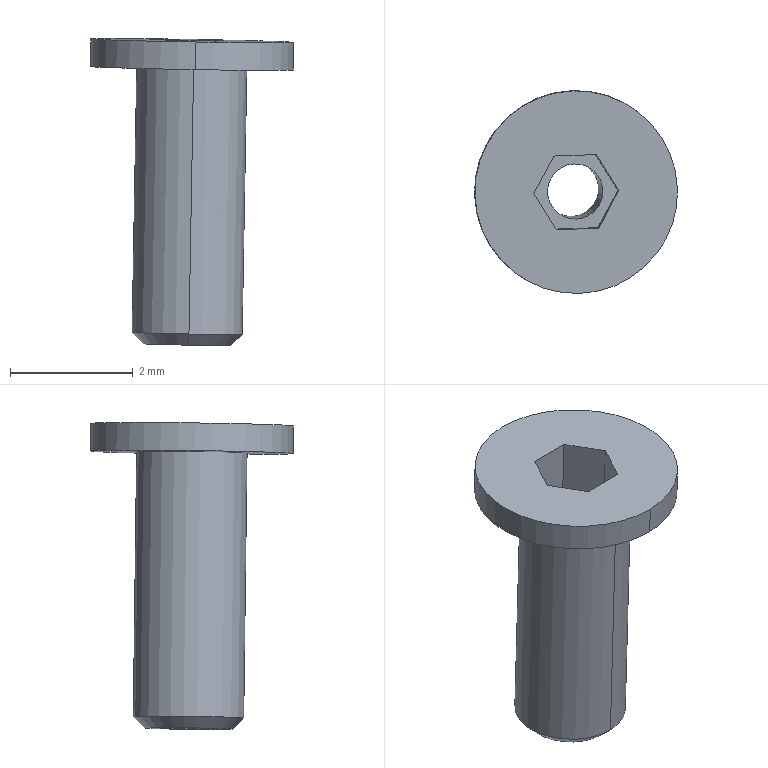Component | SolidWorks | 00-VacuumSuctionCupAssembly-1_10-SuctionCupAirHoleScrew-12 | 1 solid | 18 faces | box 3.31 x 3.31 x 5 mm | volume 12 mm3 | plane 10 | cylinder 6 | cone 2 | commonest cylinder face diameters 0.9 x2 1.8 x2 3.3 x2
STEP:
#1=COLOUR_RGB('',0.7922,0.8196,0.9333);
#2=FILL_AREA_STYLE_COLOUR('',#1);
#3=FILL_AREA_STYLE('',(#2));
#4=SURFACE_STYLE_FILL_AREA(#3);
#5=SURFACE_SIDE_STYLE('',(#4));
#6=SURFACE_STYLE_USAGE(.BOTH.,#5);
#7=PRESENTATION_STYLE_ASSIGNMENT((#6));
#8=CARTESIAN_POINT('',(2.26,5.23,2.116));
#9=VERTEX_POINT('',#8);
#10=CARTESIAN_POINT('',(2.258,5.286,2.117));
#11=VERTEX_POINT('',#10);
#12=CARTESIAN_POINT('',(2.259,5.258,2.116));
#13=DIRECTION('',(-0.01745,0.01259,-0.9998));
#14=DIRECTION('',(0.03309,-0.9994,-0.01316));
#15=AXIS2_PLACEMENT_3D('',#12,#13,#14);
#16=CIRCLE('',#15,0.02819);
#17=EDGE_CURVE('',#9,#11,#16,.T.);
#18=ORIENTED_EDGE('',*,*,#17,.F.);
#19=CARTESIAN_POINT('',(2.26,5.223,2.123));
#20=VERTEX_POINT('',#19);
#21=CARTESIAN_POINT('',(2.26,5.23,2.116));
#22=DIRECTION('',(0.03574,-0.7156,0.6976));
#23=VECTOR('',#22,39.37);
#24=LINE('',#21,#23);
#25=EDGE_CURVE('',#9,#20,#24,.T.);
#26=ORIENTED_EDGE('',*,*,#25,.T.);
#27=CARTESIAN_POINT('',(2.258,5.293,2.124));
#28=VERTEX_POINT('',#27);
#29=CARTESIAN_POINT('',(2.259,5.258,2.124));
#30=DIRECTION('',(0.01745,-0.01259,0.9998));
#31=DIRECTION('',(0.03309,-0.9994,-0.01316));
#32=AXIS2_PLACEMENT_3D('',#29,#30,#31);
#33=CIRCLE('',#32,0.03543);
#34=EDGE_CURVE('',#28,#20,#33,.T.);
#35=ORIENTED_EDGE('',*,*,#34,.F.);
#36=CARTESIAN_POINT('',(2.258,5.286,2.117));
#37=DIRECTION('',(-0.01106,0.6978,0.7162));
#38=VECTOR('',#37,39.37);
#39=LINE('',#36,#38);
#40=EDGE_CURVE('',#11,#28,#39,.T.);
#41=ORIENTED_EDGE('',*,*,#40,.F.);
#42=EDGE_LOOP('',(#18,#26,#35,#41));
#43=FACE_OUTER_BOUND('',#42,.T.);
#44=CARTESIAN_POINT('',(2.259,5.258,2.116));
#45=DIRECTION('',(0.01745,-0.01259,0.9998));
#46=DIRECTION('',(-0.03309,0.9994,0.01316));
#47=AXIS2_PLACEMENT_3D('',#44,#45,#46);
#48=CONICAL_SURFACE('',#47,0.02819,0.7854);
#49=ADVANCED_FACE('',(#43),#48,.T.);
#50=CARTESIAN_POINT('',(2.262,5.238,2.276));
#51=VERTEX_POINT('',#50);
#52=CARTESIAN_POINT('',(2.261,5.274,2.276));
#53=VERTEX_POINT('',#52);
#54=CARTESIAN_POINT('',(2.262,5.256,2.276));
#55=DIRECTION('',(0.01745,-0.01259,0.9998));
#56=DIRECTION('',(-0.03309,0.9994,0.01316));
#57=AXIS2_PLACEMENT_3D('',#54,#55,#56);
#58=CIRCLE('',#57,0.01772);
#59=EDGE_CURVE('',#51,#53,#58,.T.);
#60=ORIENTED_EDGE('',*,*,#59,.T.);
#61=CARTESIAN_POINT('',(2.258,5.276,2.117));
#62=VERTEX_POINT('',#61);
#63=CARTESIAN_POINT('',(2.258,5.276,2.117));
#64=DIRECTION('',(-0.01745,0.01259,-0.9998));
#65=VECTOR('',#64,39.37);
#66=LINE('',#63,#65);
#67=EDGE_CURVE('',#53,#62,#66,.T.);
#68=ORIENTED_EDGE('',*,*,#67,.T.);
#69=CARTESIAN_POINT('',(2.26,5.24,2.116));
#70=VERTEX_POINT('',#69);
#71=CARTESIAN_POINT('',(2.259,5.258,2.116));
#72=DIRECTION('',(-0.01745,0.01259,-0.9998));
#73=DIRECTION('',(0.03309,-0.9994,-0.01316));
#74=AXIS2_PLACEMENT_3D('',#71,#72,#73);
#75=CIRCLE('',#74,0.01772);
#76=EDGE_CURVE('',#62,#70,#75,.T.);
#77=ORIENTED_EDGE('',*,*,#76,.T.);
#78=CARTESIAN_POINT('',(2.26,5.24,2.116));
#79=DIRECTION('',(-0.01745,0.01259,-0.9998));
#80=VECTOR('',#79,39.37);
#81=LINE('',#78,#80);
#82=EDGE_CURVE('',#51,#70,#81,.T.);
#83=ORIENTED_EDGE('',*,*,#82,.F.);
#84=EDGE_LOOP('',(#60,#68,#77,#83));
#85=FACE_OUTER_BOUND('',#84,.T.);
#86=CARTESIAN_POINT('',(2.259,5.258,2.116));
#87=DIRECTION('',(-0.01745,0.01259,-0.9998));
#88=DIRECTION('',(0.03309,-0.9994,-0.01316));
#89=AXIS2_PLACEMENT_3D('',#86,#87,#88);
#90=CYLINDRICAL_SURFACE('',#89,0.01772);
#91=ADVANCED_FACE('',(#85),#90,.F.);
#92=ORIENTED_EDGE('',*,*,#34,.T.);
#93=CARTESIAN_POINT('',(2.263,5.221,2.293));
#94=VERTEX_POINT('',#93);
#95=CARTESIAN_POINT('',(2.26,5.223,2.116));
#96=DIRECTION('',(0.01745,-0.01259,0.9998));
#97=VECTOR('',#96,39.37);
#98=LINE('',#95,#97);
#99=EDGE_CURVE('',#20,#94,#98,.T.);
#100=ORIENTED_EDGE('',*,*,#99,.T.);
#101=CARTESIAN_POINT('',(2.261,5.291,2.294));
#102=VERTEX_POINT('',#101);
#103=CARTESIAN_POINT('',(2.262,5.256,2.293));
#104=DIRECTION('',(-0.01745,0.01259,-0.9998));
#105=DIRECTION('',(0.03309,-0.9994,-0.01316));
#106=AXIS2_PLACEMENT_3D('',#103,#104,#105);
#107=CIRCLE('',#106,0.03543);
#108=EDGE_CURVE('',#94,#102,#107,.T.);
#109=ORIENTED_EDGE('',*,*,#108,.T.);
#110=CARTESIAN_POINT('',(2.258,5.294,2.117));
#111=DIRECTION('',(0.01745,-0.01259,0.9998));
#112=VECTOR('',#111,39.37);
#113=LINE('',#110,#112);
#114=EDGE_CURVE('',#28,#102,#113,.T.);
#115=ORIENTED_EDGE('',*,*,#114,.F.);
#116=EDGE_LOOP('',(#92,#100,#109,#115));
#117=FACE_OUTER_BOUND('',#116,.T.);
#118=CARTESIAN_POINT('',(2.259,5.258,2.116));
#119=DIRECTION('',(0.01745,-0.01259,0.9998));
#120=DIRECTION('',(-0.03309,0.9994,0.01316));
#121=AXIS2_PLACEMENT_3D('',#118,#119,#120);
#122=CYLINDRICAL_SURFACE('',#121,0.03543);
#123=ADVANCED_FACE('',(#117),#122,.T.);
#124=CARTESIAN_POINT('',(2.26,5.321,2.294));
#125=VERTEX_POINT('',#124);
#126=CARTESIAN_POINT('',(2.264,5.191,2.293));
#127=VERTEX_POINT('',#126);
#128=CARTESIAN_POINT('',(2.262,5.256,2.293));
#129=DIRECTION('',(0.01745,-0.01259,0.9998));
#130=DIRECTION('',(-0.03309,0.9994,0.01316));
#131=AXIS2_PLACEMENT_3D('',#128,#129,#130);
#132=CIRCLE('',#131,0.06496);
#133=EDGE_CURVE('',#125,#127,#132,.T.);
#134=ORIENTED_EDGE('',*,*,#133,.T.);
#135=CARTESIAN_POINT('',(2.264,5.191,2.31));
#136=VERTEX_POINT('',#135);
#137=CARTESIAN_POINT('',(2.264,5.191,2.293));
#138=DIRECTION('',(0.01745,-0.01259,0.9998));
#139=VECTOR('',#138,39.37);
#140=LINE('',#137,#139);
#141=EDGE_CURVE('',#127,#136,#140,.T.);
#142=ORIENTED_EDGE('',*,*,#141,.T.);
#143=CARTESIAN_POINT('',(2.26,5.321,2.312));
#144=VERTEX_POINT('',#143);
#145=CARTESIAN_POINT('',(2.262,5.256,2.311));
#146=DIRECTION('',(0.01745,-0.01259,0.9998));
#147=DIRECTION('',(-0.03309,0.9994,0.01316));
#148=AXIS2_PLACEMENT_3D('',#145,#146,#147);
#149=CIRCLE('',#148,0.06496);
#150=EDGE_CURVE('',#144,#136,#149,.T.);
#151=ORIENTED_EDGE('',*,*,#150,.F.);
#152=CARTESIAN_POINT('',(2.26,5.321,2.294));
#153=DIRECTION('',(0.01745,-0.01259,0.9998));
#154=VECTOR('',#153,39.37);
#155=LINE('',#152,#154);
#156=EDGE_CURVE('',#125,#144,#155,.T.);
#157=ORIENTED_EDGE('',*,*,#156,.F.);
#158=EDGE_LOOP('',(#134,#142,#151,#157));
#159=FACE_OUTER_BOUND('',#158,.T.);
#160=CARTESIAN_POINT('',(2.262,5.256,2.293));
#161=DIRECTION('',(0.01745,-0.01259,0.9998));
#162=DIRECTION('',(-0.03309,0.9994,0.01316));
#163=AXIS2_PLACEMENT_3D('',#160,#161,#162);
#164=CYLINDRICAL_SURFACE('',#163,0.06496);
#165=ADVANCED_FACE('',(#159),#164,.T.);
#166=ORIENTED_EDGE('',*,*,#133,.F.);
#167=CARTESIAN_POINT('',(2.262,5.256,2.293));
#168=DIRECTION('',(0.01745,-0.01259,0.9998));
#169=DIRECTION('',(-0.03309,0.9994,0.01316));
#170=AXIS2_PLACEMENT_3D('',#167,#168,#169);
#171=CIRCLE('',#170,0.06496);
#172=EDGE_CURVE('',#127,#125,#171,.T.);
#173=ORIENTED_EDGE('',*,*,#172,.F.);
#174=EDGE_LOOP('',(#166,#173));
#175=FACE_OUTER_BOUND('',#174,.T.);
#176=CARTESIAN_POINT('',(2.262,5.256,2.293));
#177=DIRECTION('',(-0.01745,0.01259,-0.9998));
#178=DIRECTION('',(0.03309,-0.9994,-0.01316));
#179=AXIS2_PLACEMENT_3D('',#176,#177,#178);
#180=CIRCLE('',#179,0.03543);
#181=EDGE_CURVE('',#102,#94,#180,.T.);
#182=ORIENTED_EDGE('',*,*,#181,.F.);
#183=ORIENTED_EDGE('',*,*,#108,.F.);
#184=EDGE_LOOP('',(#182,#183));
#185=FACE_BOUND('',#184,.T.);
#186=CARTESIAN_POINT('',(2.197,5.254,2.295));
#187=DIRECTION('',(-0.01745,0.01259,-0.9998));
#188=DIRECTION('',(0.03309,-0.9994,-0.01316));
#189=AXIS2_PLACEMENT_3D('',#186,#187,#188);
#190=PLANE('',#189);
#191=ADVANCED_FACE('',(#175,#185),#190,.T.);
#192=ORIENTED_EDGE('',*,*,#141,.F.);
#193=ORIENTED_EDGE('',*,*,#172,.T.);
#194=ORIENTED_EDGE('',*,*,#156,.T.);
#195=CARTESIAN_POINT('',(2.262,5.256,2.311));
#196=DIRECTION('',(0.01745,-0.01259,0.9998));
#197=DIRECTION('',(-0.03309,0.9994,0.01316));
#198=AXIS2_PLACEMENT_3D('',#195,#196,#197);
#199=CIRCLE('',#198,0.06496);
#200=EDGE_CURVE('',#136,#144,#199,.T.);
#201=ORIENTED_EDGE('',*,*,#200,.F.);
#202=EDGE_LOOP('',(#192,#193,#194,#201));
#203=FACE_OUTER_BOUND('',#202,.T.);
#204=CARTESIAN_POINT('',(2.262,5.256,2.293));
#205=DIRECTION('',(0.01745,-0.01259,0.9998));
#206=DIRECTION('',(-0.03309,0.9994,0.01316));
#207=AXIS2_PLACEMENT_3D('',#204,#205,#206);
#208=CYLINDRICAL_SURFACE('',#207,0.06496);
#209=ADVANCED_FACE('',(#203),#208,.T.);
#210=CARTESIAN_POINT('',(2.249,5.232,2.311));
#211=VERTEX_POINT('',#210);
#212=CARTESIAN_POINT('',(2.277,5.233,2.311));
#213=VERTEX_POINT('',#212);
#214=CARTESIAN_POINT('',(2.249,5.232,2.311));
#215=DIRECTION('',(0.9993,0.03332,-0.01702));
#216=VECTOR('',#215,39.37);
#217=LINE('',#214,#216);
#218=EDGE_CURVE('',#211,#213,#217,.T.);
#219=ORIENTED_EDGE('',*,*,#218,.F.);
#220=CARTESIAN_POINT('',(2.235,5.255,2.312));
#221=VERTEX_POINT('',#220);
#222=CARTESIAN_POINT('',(2.235,5.255,2.312));
#223=DIRECTION('',(0.5283,-0.8488,-0.01991));
#224=VECTOR('',#223,39.37);
#225=LINE('',#222,#224);
#226=EDGE_CURVE('',#221,#211,#225,.T.);
#227=ORIENTED_EDGE('',*,*,#226,.F.);
#228=CARTESIAN_POINT('',(2.248,5.279,2.312));
#229=VERTEX_POINT('',#228);
#230=CARTESIAN_POINT('',(2.248,5.279,2.312));
#231=DIRECTION('',(-0.471,-0.8821,-0.002886));
#232=VECTOR('',#231,39.37);
#233=LINE('',#230,#232);
#234=EDGE_CURVE('',#229,#221,#233,.T.);
#235=ORIENTED_EDGE('',*,*,#234,.F.);
#236=CARTESIAN_POINT('',(2.275,5.28,2.311));
#237=VERTEX_POINT('',#236);
#238=CARTESIAN_POINT('',(2.275,5.28,2.311));
#239=DIRECTION('',(-0.9993,-0.03332,0.01702));
#240=VECTOR('',#239,39.37);
#241=LINE('',#238,#240);
#242=EDGE_CURVE('',#237,#229,#241,.T.);
#243=ORIENTED_EDGE('',*,*,#242,.F.);
#244=CARTESIAN_POINT('',(2.29,5.257,2.311));
#245=VERTEX_POINT('',#244);
#246=CARTESIAN_POINT('',(2.29,5.257,2.311));
#247=DIRECTION('',(-0.5283,0.8488,0.01991));
#248=VECTOR('',#247,39.37);
#249=LINE('',#246,#248);
#250=EDGE_CURVE('',#245,#237,#249,.T.);
#251=ORIENTED_EDGE('',*,*,#250,.F.);
#252=CARTESIAN_POINT('',(2.277,5.233,2.311));
#253=DIRECTION('',(0.471,0.8821,0.002886));
#254=VECTOR('',#253,39.37);
#255=LINE('',#252,#254);
#256=EDGE_CURVE('',#213,#245,#255,.T.);
#257=ORIENTED_EDGE('',*,*,#256,.F.);
#258=EDGE_LOOP('',(#219,#227,#235,#243,#251,#257));
#259=FACE_BOUND('',#258,.T.);
#260=ORIENTED_EDGE('',*,*,#150,.T.);
#261=ORIENTED_EDGE('',*,*,#200,.T.);
#262=EDGE_LOOP('',(#260,#261));
#263=FACE_OUTER_BOUND('',#262,.T.);
#264=CARTESIAN_POINT('',(2.262,5.256,2.311));
#265=DIRECTION('',(0.01745,-0.01259,0.9998));
#266=DIRECTION('',(-0.03309,0.9994,0.01316));
#267=AXIS2_PLACEMENT_3D('',#264,#265,#266);
#268=PLANE('',#267);
#269=ADVANCED_FACE('',(#259,#263),#268,.T.);
#270=ORIENTED_EDGE('',*,*,#99,.F.);
#271=CARTESIAN_POINT('',(2.259,5.258,2.124));
#272=DIRECTION('',(0.01745,-0.01259,0.9998));
#273=DIRECTION('',(0.03309,-0.9994,-0.01316));
#274=AXIS2_PLACEMENT_3D('',#271,#272,#273);
#275=CIRCLE('',#274,0.03543);
#276=EDGE_CURVE('',#20,#28,#275,.T.);
#277=ORIENTED_EDGE('',*,*,#276,.T.);
#278=ORIENTED_EDGE('',*,*,#114,.T.);
#279=ORIENTED_EDGE('',*,*,#181,.T.);
#280=EDGE_LOOP('',(#270,#277,#278,#279));
#281=FACE_OUTER_BOUND('',#280,.T.);
#282=CARTESIAN_POINT('',(2.259,5.258,2.116));
#283=DIRECTION('',(0.01745,-0.01259,0.9998));
#284=DIRECTION('',(-0.03309,0.9994,0.01316));
#285=AXIS2_PLACEMENT_3D('',#282,#283,#284);
#286=CYLINDRICAL_SURFACE('',#285,0.03543);
#287=ADVANCED_FACE('',(#281),#286,.T.);
#288=CARTESIAN_POINT('',(2.259,5.258,2.116));
#289=DIRECTION('',(-0.01745,0.01259,-0.9998));
#290=DIRECTION('',(0.03309,-0.9994,-0.01316));
#291=AXIS2_PLACEMENT_3D('',#288,#289,#290);
#292=CIRCLE('',#291,0.02819);
#293=EDGE_CURVE('',#11,#9,#292,.T.);
#294=ORIENTED_EDGE('',*,*,#293,.T.);
#295=ORIENTED_EDGE('',*,*,#17,.T.);
#296=EDGE_LOOP('',(#294,#295));
#297=FACE_OUTER_BOUND('',#296,.T.);
#298=CARTESIAN_POINT('',(2.259,5.258,2.116));
#299=DIRECTION('',(-0.01745,0.01259,-0.9998));
#300=DIRECTION('',(0.03309,-0.9994,-0.01316));
#301=AXIS2_PLACEMENT_3D('',#298,#299,#300);
#302=CIRCLE('',#301,0.01772);
#303=EDGE_CURVE('',#70,#62,#302,.T.);
#304=ORIENTED_EDGE('',*,*,#303,.F.);
#305=ORIENTED_EDGE('',*,*,#76,.F.);
#306=EDGE_LOOP('',(#304,#305));
#307=FACE_BOUND('',#306,.T.);
#308=CARTESIAN_POINT('',(2.259,5.258,2.116));
#309=DIRECTION('',(-0.01745,0.01259,-0.9998));
#310=DIRECTION('',(0.03309,-0.9994,-0.01316));
#311=AXIS2_PLACEMENT_3D('',#308,#309,#310);
#312=PLANE('',#311);
#313=ADVANCED_FACE('',(#297,#307),#312,.T.);
#314=ORIENTED_EDGE('',*,*,#218,.T.);
#315=CARTESIAN_POINT('',(2.276,5.233,2.275));
#316=VERTEX_POINT('',#315);
#317=CARTESIAN_POINT('',(2.276,5.233,2.275));
#318=DIRECTION('',(0.01745,-0.01259,0.9998));
#319=VECTOR('',#318,39.37);
#320=LINE('',#317,#319);
#321=EDGE_CURVE('',#316,#213,#320,.T.);
#322=ORIENTED_EDGE('',*,*,#321,.F.);
#323=CARTESIAN_POINT('',(2.249,5.232,2.276));
#324=VERTEX_POINT('',#323);
#325=CARTESIAN_POINT('',(2.249,5.232,2.276));
#326=DIRECTION('',(0.9993,0.03332,-0.01702));
#327=VECTOR('',#326,39.37);
#328=LINE('',#325,#327);
#329=EDGE_CURVE('',#324,#316,#328,.T.);
#330=ORIENTED_EDGE('',*,*,#329,.F.);
#331=CARTESIAN_POINT('',(2.249,5.232,2.276));
#332=DIRECTION('',(0.01745,-0.01259,0.9998));
#333=VECTOR('',#332,39.37);
#334=LINE('',#331,#333);
#335=EDGE_CURVE('',#324,#211,#334,.T.);
#336=ORIENTED_EDGE('',*,*,#335,.T.);
#337=EDGE_LOOP('',(#314,#322,#330,#336));
#338=FACE_OUTER_BOUND('',#337,.T.);
#339=CARTESIAN_POINT('',(2.249,5.232,2.276));
#340=DIRECTION('',(0.03309,-0.9994,-0.01316));
#341=DIRECTION('',(-0.9993,-0.03332,0.01702));
#342=AXIS2_PLACEMENT_3D('',#339,#340,#341);
#343=PLANE('',#342);
#344=ADVANCED_FACE('',(#338),#343,.F.);
#345=ORIENTED_EDGE('',*,*,#226,.T.);
#346=ORIENTED_EDGE('',*,*,#335,.F.);
#347=CARTESIAN_POINT('',(2.234,5.255,2.276));
#348=VERTEX_POINT('',#347);
#349=CARTESIAN_POINT('',(2.234,5.255,2.276));
#350=DIRECTION('',(0.5283,-0.8488,-0.01991));
#351=VECTOR('',#350,39.37);
#352=LINE('',#349,#351);
#353=EDGE_CURVE('',#348,#324,#352,.T.);
#354=ORIENTED_EDGE('',*,*,#353,.F.);
#355=CARTESIAN_POINT('',(2.234,5.255,2.276));
#356=DIRECTION('',(0.01745,-0.01259,0.9998));
#357=VECTOR('',#356,39.37);
#358=LINE('',#355,#357);
#359=EDGE_CURVE('',#348,#221,#358,.T.);
#360=ORIENTED_EDGE('',*,*,#359,.T.);
#361=EDGE_LOOP('',(#345,#346,#354,#360));
#362=FACE_OUTER_BOUND('',#361,.T.);
#363=CARTESIAN_POINT('',(2.234,5.255,2.276));
#364=DIRECTION('',(-0.8489,-0.5285,0.008162));
#365=DIRECTION('',(-0.5283,0.8488,0.01991));
#366=AXIS2_PLACEMENT_3D('',#363,#364,#365);
#367=PLANE('',#366);
#368=ADVANCED_FACE('',(#362),#367,.F.);
#369=ORIENTED_EDGE('',*,*,#234,.T.);
#370=ORIENTED_EDGE('',*,*,#359,.F.);
#371=CARTESIAN_POINT('',(2.247,5.279,2.276));
#372=VERTEX_POINT('',#371);
#373=CARTESIAN_POINT('',(2.247,5.279,2.276));
#374=DIRECTION('',(-0.471,-0.8821,-0.002886));
#375=VECTOR('',#374,39.37);
#376=LINE('',#373,#375);
#377=EDGE_CURVE('',#372,#348,#376,.T.);
#378=ORIENTED_EDGE('',*,*,#377,.F.);
#379=CARTESIAN_POINT('',(2.247,5.279,2.276));
#380=DIRECTION('',(0.01745,-0.01259,0.9998));
#381=VECTOR('',#380,39.37);
#382=LINE('',#379,#381);
#383=EDGE_CURVE('',#372,#229,#382,.T.);
#384=ORIENTED_EDGE('',*,*,#383,.T.);
#385=EDGE_LOOP('',(#369,#370,#378,#384));
#386=FACE_OUTER_BOUND('',#385,.T.);
#387=CARTESIAN_POINT('',(2.247,5.279,2.276));
#388=DIRECTION('',(-0.882,0.4708,0.02132));
#389=DIRECTION('',(0.471,0.8821,0.002886));
#390=AXIS2_PLACEMENT_3D('',#387,#388,#389);
#391=PLANE('',#390);
#392=ADVANCED_FACE('',(#386),#391,.F.);
#393=ORIENTED_EDGE('',*,*,#242,.T.);
#394=ORIENTED_EDGE('',*,*,#383,.F.);
#395=CARTESIAN_POINT('',(2.275,5.28,2.276));
#396=VERTEX_POINT('',#395);
#397=CARTESIAN_POINT('',(2.275,5.28,2.276));
#398=DIRECTION('',(-0.9993,-0.03332,0.01702));
#399=VECTOR('',#398,39.37);
#400=LINE('',#397,#399);
#401=EDGE_CURVE('',#396,#372,#400,.T.);
#402=ORIENTED_EDGE('',*,*,#401,.F.);
#403=CARTESIAN_POINT('',(2.275,5.28,2.276));
#404=DIRECTION('',(0.01745,-0.01259,0.9998));
#405=VECTOR('',#404,39.37);
#406=LINE('',#403,#405);
#407=EDGE_CURVE('',#396,#237,#406,.T.);
#408=ORIENTED_EDGE('',*,*,#407,.T.);
#409=EDGE_LOOP('',(#393,#394,#402,#408));
#410=FACE_OUTER_BOUND('',#409,.T.);
#411=CARTESIAN_POINT('',(2.275,5.28,2.276));
#412=DIRECTION('',(-0.03309,0.9994,0.01316));
#413=DIRECTION('',(0.9993,0.03332,-0.01702));
#414=AXIS2_PLACEMENT_3D('',#411,#412,#413);
#415=PLANE('',#414);
#416=ADVANCED_FACE('',(#410),#415,.F.);
#417=ORIENTED_EDGE('',*,*,#250,.T.);
#418=ORIENTED_EDGE('',*,*,#407,.F.);
#419=CARTESIAN_POINT('',(2.289,5.257,2.275));
#420=VERTEX_POINT('',#419);
#421=CARTESIAN_POINT('',(2.289,5.257,2.275));
#422=DIRECTION('',(-0.5283,0.8488,0.01991));
#423=VECTOR('',#422,39.37);
#424=LINE('',#421,#423);
#425=EDGE_CURVE('',#420,#396,#424,.T.);
#426=ORIENTED_EDGE('',*,*,#425,.F.);
#427=CARTESIAN_POINT('',(2.289,5.257,2.275));
#428=DIRECTION('',(0.01745,-0.01259,0.9998));
#429=VECTOR('',#428,39.37);
#430=LINE('',#427,#429);
#431=EDGE_CURVE('',#420,#245,#430,.T.);
#432=ORIENTED_EDGE('',*,*,#431,.T.);
#433=EDGE_LOOP('',(#417,#418,#426,#432));
#434=FACE_OUTER_BOUND('',#433,.T.);
#435=CARTESIAN_POINT('',(2.289,5.257,2.275));
#436=DIRECTION('',(0.8489,0.5285,-0.008162));
#437=DIRECTION('',(0.5283,-0.8488,-0.01991));
#438=AXIS2_PLACEMENT_3D('',#435,#436,#437);
#439=PLANE('',#438);
#440=ADVANCED_FACE('',(#434),#439,.F.);
#441=ORIENTED_EDGE('',*,*,#256,.T.);
#442=ORIENTED_EDGE('',*,*,#431,.F.);
#443=CARTESIAN_POINT('',(2.276,5.233,2.275));
#444=DIRECTION('',(0.471,0.8821,0.002886));
#445=VECTOR('',#444,39.37);
#446=LINE('',#443,#445);
#447=EDGE_CURVE('',#316,#420,#446,.T.);
#448=ORIENTED_EDGE('',*,*,#447,.F.);
#449=ORIENTED_EDGE('',*,*,#321,.T.);
#450=EDGE_LOOP('',(#441,#442,#448,#449));
#451=FACE_OUTER_BOUND('',#450,.T.);
#452=CARTESIAN_POINT('',(2.276,5.233,2.275));
#453=DIRECTION('',(0.882,-0.4708,-0.02132));
#454=DIRECTION('',(-0.471,-0.8821,-0.002886));
#455=AXIS2_PLACEMENT_3D('',#452,#453,#454);
#456=PLANE('',#455);
#457=ADVANCED_FACE('',(#451),#456,.F.);
#458=ORIENTED_EDGE('',*,*,#59,.F.);
#459=CARTESIAN_POINT('',(2.262,5.256,2.276));
#460=DIRECTION('',(0.01745,-0.01259,0.9998));
#461=DIRECTION('',(-0.03309,0.9994,0.01316));
#462=AXIS2_PLACEMENT_3D('',#459,#460,#461);
#463=CIRCLE('',#462,0.01772);
#464=EDGE_CURVE('',#53,#51,#463,.T.);
#465=ORIENTED_EDGE('',*,*,#464,.F.);
#466=EDGE_LOOP('',(#458,#465));
#467=FACE_BOUND('',#466,.T.);
#468=ORIENTED_EDGE('',*,*,#329,.T.);
#469=ORIENTED_EDGE('',*,*,#447,.T.);
#470=ORIENTED_EDGE('',*,*,#425,.T.);
#471=ORIENTED_EDGE('',*,*,#401,.T.);
#472=ORIENTED_EDGE('',*,*,#377,.T.);
#473=ORIENTED_EDGE('',*,*,#353,.T.);
#474=EDGE_LOOP('',(#468,#469,#470,#471,#472,#473));
#475=FACE_OUTER_BOUND('',#474,.T.);
#476=CARTESIAN_POINT('',(2.262,5.256,2.276));
#477=DIRECTION('',(0.01745,-0.01259,0.9998));
#478=DIRECTION('',(-0.03309,0.9994,0.01316));
#479=AXIS2_PLACEMENT_3D('',#476,#477,#478);
#480=PLANE('',#479);
#481=ADVANCED_FACE('',(#467,#475),#480,.T.);
#482=ORIENTED_EDGE('',*,*,#67,.F.);
#483=ORIENTED_EDGE('',*,*,#464,.T.);
#484=ORIENTED_EDGE('',*,*,#82,.T.);
#485=ORIENTED_EDGE('',*,*,#303,.T.);
#486=EDGE_LOOP('',(#482,#483,#484,#485));
#487=FACE_OUTER_BOUND('',#486,.T.);
#488=CARTESIAN_POINT('',(2.259,5.258,2.116));
#489=DIRECTION('',(-0.01745,0.01259,-0.9998));
#490=DIRECTION('',(0.03309,-0.9994,-0.01316));
#491=AXIS2_PLACEMENT_3D('',#488,#489,#490);
#492=CYLINDRICAL_SURFACE('',#491,0.01772);
#493=ADVANCED_FACE('',(#487),#492,.F.);
#494=ORIENTED_EDGE('',*,*,#25,.F.);
#495=ORIENTED_EDGE('',*,*,#293,.F.);
#496=ORIENTED_EDGE('',*,*,#40,.T.);
#497=ORIENTED_EDGE('',*,*,#276,.F.);
#498=EDGE_LOOP('',(#494,#495,#496,#497));
#499=FACE_OUTER_BOUND('',#498,.T.);
#500=CARTESIAN_POINT('',(2.259,5.258,2.116));
#501=DIRECTION('',(0.01745,-0.01259,0.9998));
#502=DIRECTION('',(-0.03309,0.9994,0.01316));
#503=AXIS2_PLACEMENT_3D('',#500,#501,#502);
#504=CONICAL_SURFACE('',#503,0.02819,0.7854);
#505=ADVANCED_FACE('',(#499),#504,.T.);
#506=CLOSED_SHELL('',(#49,#91,#123,#165,#191,#209,#269,#287,#313,#344,#368,#392,#416,#440,#457,#481,#493,#505));
#507=MANIFOLD_SOLID_BREP('',#506);
#508=STYLED_ITEM('',(#7),#507);
#509=(LENGTH_UNIT()NAMED_UNIT(*)SI_UNIT($,.METRE.));
#510=LENGTH_MEASURE_WITH_UNIT(LENGTH_MEASURE(0.0254),#509);
#511=DIMENSIONAL_EXPONENTS(1.,0.,0.,0.,0.,0.,0.);
#512=(CONVERSION_BASED_UNIT('',#510)LENGTH_UNIT()NAMED_UNIT(#511));
#513=UNCERTAINTY_MEASURE_WITH_UNIT(LENGTH_MEASURE(0.00001),#512,'','');
#514=(NAMED_UNIT(*)PLANE_ANGLE_UNIT()SI_UNIT($,.RADIAN.));
#515=(NAMED_UNIT(*)SI_UNIT($,.STERADIAN.)SOLID_ANGLE_UNIT());
#516=(GEOMETRIC_REPRESENTATION_CONTEXT(3)GLOBAL_UNCERTAINTY_ASSIGNED_CONTEXT((#513))GLOBAL_UNIT_ASSIGNED_CONTEXT((#512,#514,#515))REPRESENTATION_CONTEXT('',''));
#517=MECHANICAL_DESIGN_GEOMETRIC_PRESENTATION_REPRESENTATION('',(#508),#516);
#518=PRESENTATION_LAYER_ASSIGNMENT('','',(#508));
#519=CARTESIAN_POINT('',(0.,0.,0.));
#520=DIRECTION('',(0.,0.,1.));
#521=DIRECTION('',(1.,0.,0.));
#522=AXIS2_PLACEMENT_3D('',#519,#520,#521);
#523=(LENGTH_UNIT()NAMED_UNIT(*)SI_UNIT($,.METRE.));
#524=LENGTH_MEASURE_WITH_UNIT(LENGTH_MEASURE(0.0254),#523);
#525=DIMENSIONAL_EXPONENTS(1.,0.,0.,0.,0.,0.,0.);
#526=(CONVERSION_BASED_UNIT('',#524)LENGTH_UNIT()NAMED_UNIT(#525));
#527=UNCERTAINTY_MEASURE_WITH_UNIT(LENGTH_MEASURE(0.00001),#526,'','');
#528=(NAMED_UNIT(*)PLANE_ANGLE_UNIT()SI_UNIT($,.RADIAN.));
#529=(NAMED_UNIT(*)SI_UNIT($,.STERADIAN.)SOLID_ANGLE_UNIT());
#530=(GEOMETRIC_REPRESENTATION_CONTEXT(3)GLOBAL_UNCERTAINTY_ASSIGNED_CONTEXT((#527))GLOBAL_UNIT_ASSIGNED_CONTEXT((#526,#528,#529))REPRESENTATION_CONTEXT('',''));
#531=ADVANCED_BREP_SHAPE_REPRESENTATION('',(#507,#522),#530);